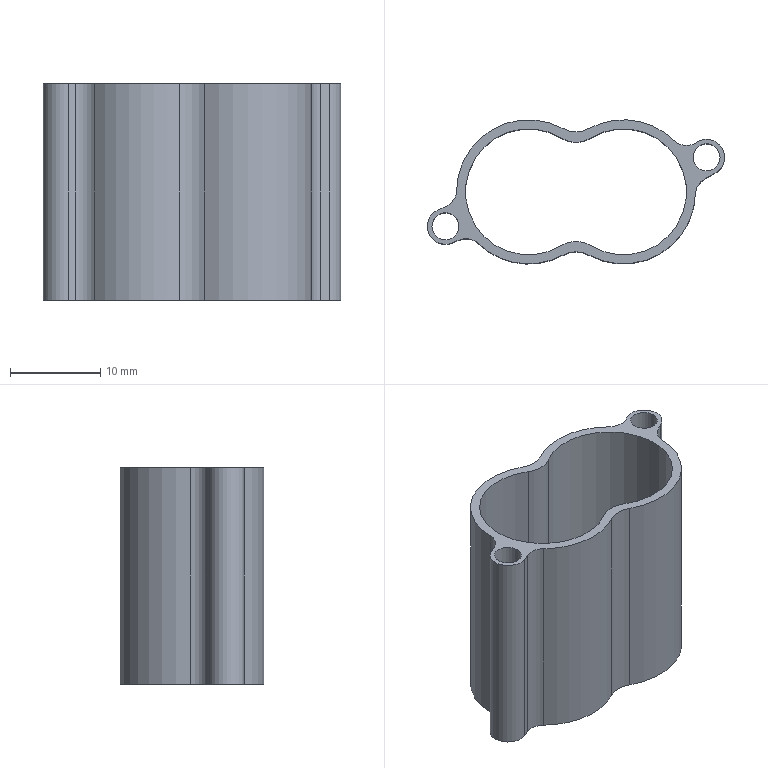Component | NX | HOUSING | 1 solid | 24 faces | volume 2073 mm3 | cylinder 18 | plane 6 | commonest cylinder face diameters 4 x6 6 x4 16 x4 14 x2 3 x2